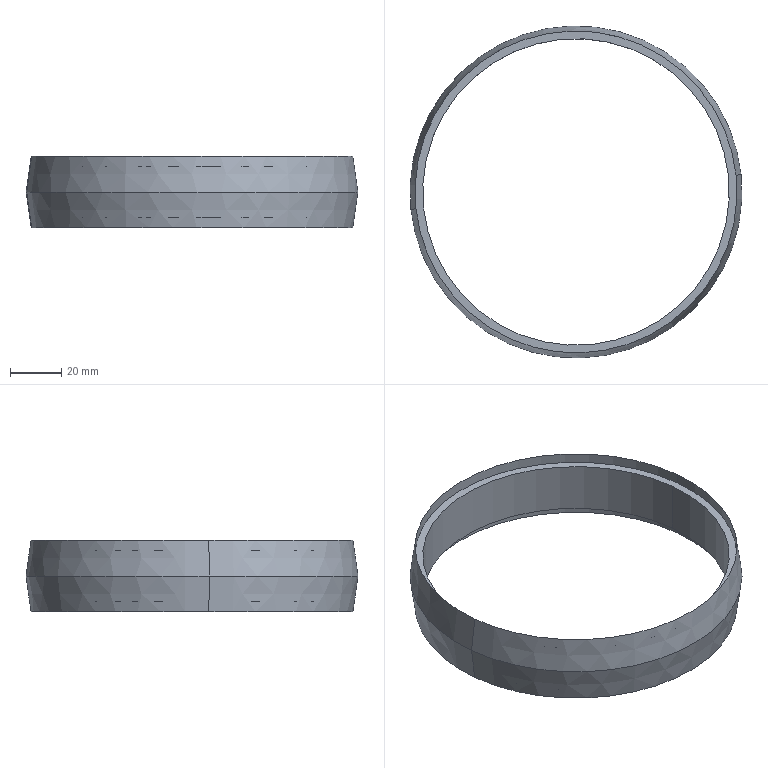Component | SolidWorks | DriveDevice-1_DriveWheelRubber-1 | 1 solid | 12 faces | box 129.97 x 129.97 x 28 mm | volume 34300 mm3 | cylinder 6 | cone 4 | plane 2 | commonest cylinder face diameters 126 x4 120 x2
build123d program:
from build123d import *


with BuildPart() as part:
    # Sketch1 → Revolve1 (revolve)
    with BuildSketch(Plane(origin=(0, 0, 0), x_dir=(0, 0, -1), z_dir=(1, 0, 0)), mode=Mode.PRIVATE) as revolve1_sk:
        Polygon((-10, 60), (10, 60), (10, 63), (14, 63), (0, 64.985), (-14, 63), (-10, 63), align=None)
    revolve(revolve1_sk.sketch.rotate(Axis((0, 0, 0), (0, 0, -1)), 90), axis=Axis((0, 0, 0), (0, 0, -1)))


solid = part.part

# Placed as in the assembly
solid = solid.moved(Location((55, 43, 51.5), (0, 0, 0)))
STEP:
#1=CARTESIAN_POINT('',(4.632,1.952,1.476));
#2=VERTEX_POINT('',#1);
#3=CARTESIAN_POINT('',(-0.3014,1.434,1.476));
#4=VERTEX_POINT('',#3);
#5=CARTESIAN_POINT('',(2.165,1.693,1.476));
#6=DIRECTION('',(0.,0.,1.));
#7=DIRECTION('',(0.9945,0.1046,0.));
#8=AXIS2_PLACEMENT_3D('',#5,#6,#7);
#9=CIRCLE('',#8,2.48);
#10=EDGE_CURVE('',#2,#4,#9,.T.);
#11=ORIENTED_EDGE('',*,*,#10,.T.);
#12=CARTESIAN_POINT('',(-0.3791,1.425,2.028));
#13=VERTEX_POINT('',#12);
#14=CARTESIAN_POINT('',(-0.3014,1.434,1.476));
#15=DIRECTION('',(-0.1396,-0.01468,0.9901));
#16=VECTOR('',#15,39.37);
#17=LINE('',#14,#16);
#18=EDGE_CURVE('',#4,#13,#17,.T.);
#19=ORIENTED_EDGE('',*,*,#18,.T.);
#20=CARTESIAN_POINT('',(4.71,1.96,2.028));
#21=VERTEX_POINT('',#20);
#22=CARTESIAN_POINT('',(2.165,1.693,2.028));
#23=DIRECTION('',(0.,0.,1.));
#24=DIRECTION('',(0.9945,0.1046,0.));
#25=AXIS2_PLACEMENT_3D('',#22,#23,#24);
#26=CIRCLE('',#25,2.558);
#27=EDGE_CURVE('',#21,#13,#26,.T.);
#28=ORIENTED_EDGE('',*,*,#27,.F.);
#29=CARTESIAN_POINT('',(4.632,1.952,1.476));
#30=DIRECTION('',(0.1396,0.01468,0.9901));
#31=VECTOR('',#30,39.37);
#32=LINE('',#29,#31);
#33=EDGE_CURVE('',#2,#21,#32,.T.);
#34=ORIENTED_EDGE('',*,*,#33,.F.);
#35=EDGE_LOOP('',(#11,#19,#28,#34));
#36=FACE_OUTER_BOUND('',#35,.T.);
#37=CARTESIAN_POINT('',(2.165,1.693,1.476));
#38=DIRECTION('',(0.,0.,1.));
#39=DIRECTION('',(0.9945,0.1046,0.));
#40=AXIS2_PLACEMENT_3D('',#37,#38,#39);
#41=CONICAL_SURFACE('',#40,2.48,0.1408);
#42=ADVANCED_FACE('',(#36),#41,.T.);
#43=CARTESIAN_POINT('',(2.165,1.693,1.476));
#44=DIRECTION('',(0.,0.,1.));
#45=DIRECTION('',(0.9945,0.1046,0.));
#46=AXIS2_PLACEMENT_3D('',#43,#44,#45);
#47=CIRCLE('',#46,2.48);
#48=EDGE_CURVE('',#4,#2,#47,.T.);
#49=ORIENTED_EDGE('',*,*,#48,.F.);
#50=CARTESIAN_POINT('',(-0.3014,1.434,1.634));
#51=VERTEX_POINT('',#50);
#52=CARTESIAN_POINT('',(-0.3014,1.434,2.028));
#53=DIRECTION('',(0.,0.,1.));
#54=VECTOR('',#53,39.37);
#55=LINE('',#52,#54);
#56=EDGE_CURVE('',#4,#51,#55,.T.);
#57=ORIENTED_EDGE('',*,*,#56,.T.);
#58=CARTESIAN_POINT('',(4.632,1.952,1.634));
#59=VERTEX_POINT('',#58);
#60=CARTESIAN_POINT('',(2.165,1.693,1.634));
#61=DIRECTION('',(0.,0.,1.));
#62=DIRECTION('',(0.9945,0.1046,0.));
#63=AXIS2_PLACEMENT_3D('',#60,#61,#62);
#64=CIRCLE('',#63,2.48);
#65=EDGE_CURVE('',#51,#59,#64,.T.);
#66=ORIENTED_EDGE('',*,*,#65,.T.);
#67=CARTESIAN_POINT('',(4.632,1.952,2.028));
#68=DIRECTION('',(0.,0.,1.));
#69=VECTOR('',#68,39.37);
#70=LINE('',#67,#69);
#71=EDGE_CURVE('',#2,#59,#70,.T.);
#72=ORIENTED_EDGE('',*,*,#71,.F.);
#73=EDGE_LOOP('',(#49,#57,#66,#72));
#74=FACE_OUTER_BOUND('',#73,.T.);
#75=CARTESIAN_POINT('',(2.165,1.693,2.028));
#76=DIRECTION('',(0.,0.,1.));
#77=DIRECTION('',(0.9945,0.1046,0.));
#78=AXIS2_PLACEMENT_3D('',#75,#76,#77);
#79=CYLINDRICAL_SURFACE('',#78,2.48);
#80=ADVANCED_FACE('',(#74),#79,.F.);
#81=CARTESIAN_POINT('',(-0.1839,1.446,1.634));
#82=VERTEX_POINT('',#81);
#83=CARTESIAN_POINT('',(4.515,1.94,1.634));
#84=VERTEX_POINT('',#83);
#85=CARTESIAN_POINT('',(2.165,1.693,1.634));
#86=DIRECTION('',(0.,0.,1.));
#87=DIRECTION('',(0.9945,0.1046,0.));
#88=AXIS2_PLACEMENT_3D('',#85,#86,#87);
#89=CIRCLE('',#88,2.362);
#90=EDGE_CURVE('',#82,#84,#89,.T.);
#91=ORIENTED_EDGE('',*,*,#90,.F.);
#92=CARTESIAN_POINT('',(-0.1839,1.446,2.421));
#93=VERTEX_POINT('',#92);
#94=CARTESIAN_POINT('',(-0.1839,1.446,2.028));
#95=DIRECTION('',(0.,0.,1.));
#96=VECTOR('',#95,39.37);
#97=LINE('',#94,#96);
#98=EDGE_CURVE('',#82,#93,#97,.T.);
#99=ORIENTED_EDGE('',*,*,#98,.T.);
#100=CARTESIAN_POINT('',(4.515,1.94,2.421));
#101=VERTEX_POINT('',#100);
#102=CARTESIAN_POINT('',(2.165,1.693,2.421));
#103=DIRECTION('',(0.,0.,1.));
#104=DIRECTION('',(0.9945,0.1046,0.));
#105=AXIS2_PLACEMENT_3D('',#102,#103,#104);
#106=CIRCLE('',#105,2.362);
#107=EDGE_CURVE('',#93,#101,#106,.T.);
#108=ORIENTED_EDGE('',*,*,#107,.T.);
#109=CARTESIAN_POINT('',(4.515,1.94,2.028));
#110=DIRECTION('',(0.,0.,1.));
#111=VECTOR('',#110,39.37);
#112=LINE('',#109,#111);
#113=EDGE_CURVE('',#84,#101,#112,.T.);
#114=ORIENTED_EDGE('',*,*,#113,.F.);
#115=EDGE_LOOP('',(#91,#99,#108,#114));
#116=FACE_OUTER_BOUND('',#115,.T.);
#117=CARTESIAN_POINT('',(2.165,1.693,2.028));
#118=DIRECTION('',(0.,0.,1.));
#119=DIRECTION('',(0.9945,0.1046,0.));
#120=AXIS2_PLACEMENT_3D('',#117,#118,#119);
#121=CYLINDRICAL_SURFACE('',#120,2.362);
#122=ADVANCED_FACE('',(#116),#121,.F.);
#123=CARTESIAN_POINT('',(-0.3014,1.434,2.421));
#124=VERTEX_POINT('',#123);
#125=CARTESIAN_POINT('',(4.632,1.952,2.421));
#126=VERTEX_POINT('',#125);
#127=CARTESIAN_POINT('',(2.165,1.693,2.421));
#128=DIRECTION('',(0.,0.,1.));
#129=DIRECTION('',(0.9945,0.1046,0.));
#130=AXIS2_PLACEMENT_3D('',#127,#128,#129);
#131=CIRCLE('',#130,2.48);
#132=EDGE_CURVE('',#124,#126,#131,.T.);
#133=ORIENTED_EDGE('',*,*,#132,.F.);
#134=CARTESIAN_POINT('',(-0.3014,1.434,2.579));
#135=VERTEX_POINT('',#134);
#136=CARTESIAN_POINT('',(-0.3014,1.434,2.028));
#137=DIRECTION('',(0.,0.,1.));
#138=VECTOR('',#137,39.37);
#139=LINE('',#136,#138);
#140=EDGE_CURVE('',#124,#135,#139,.T.);
#141=ORIENTED_EDGE('',*,*,#140,.T.);
#142=CARTESIAN_POINT('',(4.632,1.952,2.579));
#143=VERTEX_POINT('',#142);
#144=CARTESIAN_POINT('',(2.165,1.693,2.579));
#145=DIRECTION('',(0.,0.,1.));
#146=DIRECTION('',(0.9945,0.1046,0.));
#147=AXIS2_PLACEMENT_3D('',#144,#145,#146);
#148=CIRCLE('',#147,2.48);
#149=EDGE_CURVE('',#135,#143,#148,.T.);
#150=ORIENTED_EDGE('',*,*,#149,.T.);
#151=CARTESIAN_POINT('',(4.632,1.952,2.028));
#152=DIRECTION('',(0.,0.,1.));
#153=VECTOR('',#152,39.37);
#154=LINE('',#151,#153);
#155=EDGE_CURVE('',#126,#143,#154,.T.);
#156=ORIENTED_EDGE('',*,*,#155,.F.);
#157=EDGE_LOOP('',(#133,#141,#150,#156));
#158=FACE_OUTER_BOUND('',#157,.T.);
#159=CARTESIAN_POINT('',(2.165,1.693,2.028));
#160=DIRECTION('',(0.,0.,1.));
#161=DIRECTION('',(0.9945,0.1046,0.));
#162=AXIS2_PLACEMENT_3D('',#159,#160,#161);
#163=CYLINDRICAL_SURFACE('',#162,2.48);
#164=ADVANCED_FACE('',(#158),#163,.F.);
#165=CARTESIAN_POINT('',(2.165,1.693,2.579));
#166=DIRECTION('',(0.,0.,1.));
#167=DIRECTION('',(0.9945,0.1046,0.));
#168=AXIS2_PLACEMENT_3D('',#165,#166,#167);
#169=CIRCLE('',#168,2.48);
#170=EDGE_CURVE('',#143,#135,#169,.T.);
#171=ORIENTED_EDGE('',*,*,#170,.F.);
#172=CARTESIAN_POINT('',(4.71,1.96,2.028));
#173=DIRECTION('',(0.1396,0.01468,-0.9901));
#174=VECTOR('',#173,39.37);
#175=LINE('',#172,#174);
#176=EDGE_CURVE('',#143,#21,#175,.T.);
#177=ORIENTED_EDGE('',*,*,#176,.T.);
#178=ORIENTED_EDGE('',*,*,#27,.T.);
#179=CARTESIAN_POINT('',(-0.3791,1.425,2.028));
#180=DIRECTION('',(-0.1396,-0.01468,-0.9901));
#181=VECTOR('',#180,39.37);
#182=LINE('',#179,#181);
#183=EDGE_CURVE('',#135,#13,#182,.T.);
#184=ORIENTED_EDGE('',*,*,#183,.F.);
#185=EDGE_LOOP('',(#171,#177,#178,#184));
#186=FACE_OUTER_BOUND('',#185,.T.);
#187=CARTESIAN_POINT('',(2.165,1.693,2.028));
#188=DIRECTION('',(0.,0.,-1.));
#189=DIRECTION('',(-0.9945,-0.1046,0.));
#190=AXIS2_PLACEMENT_3D('',#187,#188,#189);
#191=CONICAL_SURFACE('',#190,2.558,0.1408);
#192=ADVANCED_FACE('',(#186),#191,.T.);
#193=ORIENTED_EDGE('',*,*,#176,.F.);
#194=ORIENTED_EDGE('',*,*,#149,.F.);
#195=ORIENTED_EDGE('',*,*,#183,.T.);
#196=CARTESIAN_POINT('',(2.165,1.693,2.028));
#197=DIRECTION('',(0.,0.,1.));
#198=DIRECTION('',(0.9945,0.1046,0.));
#199=AXIS2_PLACEMENT_3D('',#196,#197,#198);
#200=CIRCLE('',#199,2.558);
#201=EDGE_CURVE('',#13,#21,#200,.T.);
#202=ORIENTED_EDGE('',*,*,#201,.T.);
#203=EDGE_LOOP('',(#193,#194,#195,#202));
#204=FACE_OUTER_BOUND('',#203,.T.);
#205=CARTESIAN_POINT('',(2.165,1.693,2.028));
#206=DIRECTION('',(0.,0.,-1.));
#207=DIRECTION('',(-0.9945,-0.1046,0.));
#208=AXIS2_PLACEMENT_3D('',#205,#206,#207);
#209=CONICAL_SURFACE('',#208,2.558,0.1408);
#210=ADVANCED_FACE('',(#204),#209,.T.);
#211=ORIENTED_EDGE('',*,*,#140,.F.);
#212=CARTESIAN_POINT('',(2.165,1.693,2.421));
#213=DIRECTION('',(0.,0.,1.));
#214=DIRECTION('',(0.9945,0.1046,0.));
#215=AXIS2_PLACEMENT_3D('',#212,#213,#214);
#216=CIRCLE('',#215,2.48);
#217=EDGE_CURVE('',#126,#124,#216,.T.);
#218=ORIENTED_EDGE('',*,*,#217,.F.);
#219=ORIENTED_EDGE('',*,*,#155,.T.);
#220=ORIENTED_EDGE('',*,*,#170,.T.);
#221=EDGE_LOOP('',(#211,#218,#219,#220));
#222=FACE_OUTER_BOUND('',#221,.T.);
#223=CARTESIAN_POINT('',(2.165,1.693,2.028));
#224=DIRECTION('',(0.,0.,1.));
#225=DIRECTION('',(0.9945,0.1046,0.));
#226=AXIS2_PLACEMENT_3D('',#223,#224,#225);
#227=CYLINDRICAL_SURFACE('',#226,2.48);
#228=ADVANCED_FACE('',(#222),#227,.F.);
#229=CARTESIAN_POINT('',(2.165,1.693,2.421));
#230=DIRECTION('',(0.,0.,1.));
#231=DIRECTION('',(0.9945,0.1046,0.));
#232=AXIS2_PLACEMENT_3D('',#229,#230,#231);
#233=CIRCLE('',#232,2.362);
#234=EDGE_CURVE('',#101,#93,#233,.T.);
#235=ORIENTED_EDGE('',*,*,#234,.F.);
#236=ORIENTED_EDGE('',*,*,#107,.F.);
#237=EDGE_LOOP('',(#235,#236));
#238=FACE_BOUND('',#237,.T.);
#239=ORIENTED_EDGE('',*,*,#217,.T.);
#240=ORIENTED_EDGE('',*,*,#132,.T.);
#241=EDGE_LOOP('',(#239,#240));
#242=FACE_OUTER_BOUND('',#241,.T.);
#243=CARTESIAN_POINT('',(1.918,4.042,2.421));
#244=DIRECTION('',(0.,0.,-1.));
#245=DIRECTION('',(-0.9945,-0.1046,0.));
#246=AXIS2_PLACEMENT_3D('',#243,#244,#245);
#247=PLANE('',#246);
#248=ADVANCED_FACE('',(#238,#242),#247,.F.);
#249=ORIENTED_EDGE('',*,*,#98,.F.);
#250=CARTESIAN_POINT('',(2.165,1.693,1.634));
#251=DIRECTION('',(0.,0.,1.));
#252=DIRECTION('',(0.9945,0.1046,0.));
#253=AXIS2_PLACEMENT_3D('',#250,#251,#252);
#254=CIRCLE('',#253,2.362);
#255=EDGE_CURVE('',#84,#82,#254,.T.);
#256=ORIENTED_EDGE('',*,*,#255,.F.);
#257=ORIENTED_EDGE('',*,*,#113,.T.);
#258=ORIENTED_EDGE('',*,*,#234,.T.);
#259=EDGE_LOOP('',(#249,#256,#257,#258));
#260=FACE_OUTER_BOUND('',#259,.T.);
#261=CARTESIAN_POINT('',(2.165,1.693,2.028));
#262=DIRECTION('',(0.,0.,1.));
#263=DIRECTION('',(0.9945,0.1046,0.));
#264=AXIS2_PLACEMENT_3D('',#261,#262,#263);
#265=CYLINDRICAL_SURFACE('',#264,2.362);
#266=ADVANCED_FACE('',(#260),#265,.F.);
#267=CARTESIAN_POINT('',(2.165,1.693,1.634));
#268=DIRECTION('',(0.,0.,1.));
#269=DIRECTION('',(0.9945,0.1046,0.));
#270=AXIS2_PLACEMENT_3D('',#267,#268,#269);
#271=CIRCLE('',#270,2.48);
#272=EDGE_CURVE('',#59,#51,#271,.T.);
#273=ORIENTED_EDGE('',*,*,#272,.F.);
#274=ORIENTED_EDGE('',*,*,#65,.F.);
#275=EDGE_LOOP('',(#273,#274));
#276=FACE_OUTER_BOUND('',#275,.T.);
#277=ORIENTED_EDGE('',*,*,#255,.T.);
#278=ORIENTED_EDGE('',*,*,#90,.T.);
#279=EDGE_LOOP('',(#277,#278));
#280=FACE_BOUND('',#279,.T.);
#281=CARTESIAN_POINT('',(1.918,4.042,1.634));
#282=DIRECTION('',(0.,0.,1.));
#283=DIRECTION('',(0.9945,0.1046,0.));
#284=AXIS2_PLACEMENT_3D('',#281,#282,#283);
#285=PLANE('',#284);
#286=ADVANCED_FACE('',(#276,#280),#285,.F.);
#287=ORIENTED_EDGE('',*,*,#56,.F.);
#288=ORIENTED_EDGE('',*,*,#10,.F.);
#289=ORIENTED_EDGE('',*,*,#71,.T.);
#290=ORIENTED_EDGE('',*,*,#272,.T.);
#291=EDGE_LOOP('',(#287,#288,#289,#290));
#292=FACE_OUTER_BOUND('',#291,.T.);
#293=CARTESIAN_POINT('',(2.165,1.693,2.028));
#294=DIRECTION('',(0.,0.,1.));
#295=DIRECTION('',(0.9945,0.1046,0.));
#296=AXIS2_PLACEMENT_3D('',#293,#294,#295);
#297=CYLINDRICAL_SURFACE('',#296,2.48);
#298=ADVANCED_FACE('',(#292),#297,.F.);
#299=ORIENTED_EDGE('',*,*,#18,.F.);
#300=ORIENTED_EDGE('',*,*,#48,.T.);
#301=ORIENTED_EDGE('',*,*,#33,.T.);
#302=ORIENTED_EDGE('',*,*,#201,.F.);
#303=EDGE_LOOP('',(#299,#300,#301,#302));
#304=FACE_OUTER_BOUND('',#303,.T.);
#305=CARTESIAN_POINT('',(2.165,1.693,1.476));
#306=DIRECTION('',(0.,0.,1.));
#307=DIRECTION('',(0.9945,0.1046,0.));
#308=AXIS2_PLACEMENT_3D('',#305,#306,#307);
#309=CONICAL_SURFACE('',#308,2.48,0.1408);
#310=ADVANCED_FACE('',(#304),#309,.T.);
#311=CLOSED_SHELL('',(#42,#80,#122,#164,#192,#210,#228,#248,#266,#286,#298,#310));
#312=MANIFOLD_SOLID_BREP('',#311);
#313=CARTESIAN_POINT('',(0.,0.,0.));
#314=DIRECTION('',(0.,0.,1.));
#315=DIRECTION('',(1.,0.,0.));
#316=AXIS2_PLACEMENT_3D('',#313,#314,#315);
#317=(LENGTH_UNIT()NAMED_UNIT(*)SI_UNIT($,.METRE.));
#318=LENGTH_MEASURE_WITH_UNIT(LENGTH_MEASURE(0.0254),#317);
#319=DIMENSIONAL_EXPONENTS(1.,0.,0.,0.,0.,0.,0.);
#320=(CONVERSION_BASED_UNIT('',#318)LENGTH_UNIT()NAMED_UNIT(#319));
#321=UNCERTAINTY_MEASURE_WITH_UNIT(LENGTH_MEASURE(0.00001),#320,'','');
#322=(NAMED_UNIT(*)PLANE_ANGLE_UNIT()SI_UNIT($,.RADIAN.));
#323=(NAMED_UNIT(*)SI_UNIT($,.STERADIAN.)SOLID_ANGLE_UNIT());
#324=(GEOMETRIC_REPRESENTATION_CONTEXT(3)GLOBAL_UNCERTAINTY_ASSIGNED_CONTEXT((#321))GLOBAL_UNIT_ASSIGNED_CONTEXT((#320,#322,#323))REPRESENTATION_CONTEXT('',''));
#325=ADVANCED_BREP_SHAPE_REPRESENTATION('',(#312,#316),#324);
#326=COLOUR_RGB('',0.7922,0.8196,0.9333);
#327=FILL_AREA_STYLE_COLOUR('',#326);
#328=FILL_AREA_STYLE('',(#327));
#329=SURFACE_STYLE_FILL_AREA(#328);
#330=SURFACE_SIDE_STYLE('',(#329));
#331=SURFACE_STYLE_USAGE(.BOTH.,#330);
#332=PRESENTATION_STYLE_ASSIGNMENT((#331));
#333=STYLED_ITEM('',(#332),#312);
#334=(LENGTH_UNIT()NAMED_UNIT(*)SI_UNIT($,.METRE.));
#335=LENGTH_MEASURE_WITH_UNIT(LENGTH_MEASURE(0.0254),#334);
#336=DIMENSIONAL_EXPONENTS(1.,0.,0.,0.,0.,0.,0.);
#337=(CONVERSION_BASED_UNIT('',#335)LENGTH_UNIT()NAMED_UNIT(#336));
#338=UNCERTAINTY_MEASURE_WITH_UNIT(LENGTH_MEASURE(0.00001),#337,'','');
#339=(NAMED_UNIT(*)PLANE_ANGLE_UNIT()SI_UNIT($,.RADIAN.));
#340=(NAMED_UNIT(*)SI_UNIT($,.STERADIAN.)SOLID_ANGLE_UNIT());
#341=(GEOMETRIC_REPRESENTATION_CONTEXT(3)GLOBAL_UNCERTAINTY_ASSIGNED_CONTEXT((#338))GLOBAL_UNIT_ASSIGNED_CONTEXT((#337,#339,#340))REPRESENTATION_CONTEXT('',''));
#342=MECHANICAL_DESIGN_GEOMETRIC_PRESENTATION_REPRESENTATION('',(#333),#341);
#343=PRESENTATION_LAYER_ASSIGNMENT('','',(#333));